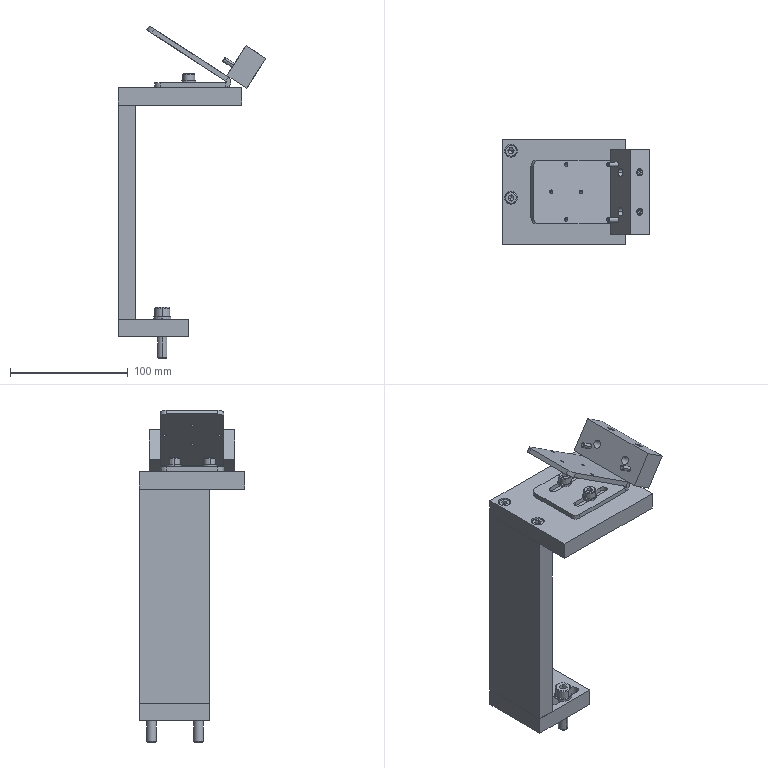Assembly | SolidWorks | mm | 21 component files | 21 solids | 450 faces | box 125.5 x 90 x 282.29 mm | volume 427306 mm3 | plane 252 | cylinder 126 | cone 72 | commonest cylinder face diameters 6 x38 10 x16 7 x12 11 x8 6.6 x8 3.3 x8 8 x8 9 x6
Bill of materials:
AdjustmentPlate | 1 |  | Bent plate bracket in one constant-thickness sheet: a flat base leg and a long inclined leg joined by a tight rounded bend, giving an acute V/stand profile. The inclined leg has four small round holes in a diamond pattern; the base leg has an elongated slot near its free end.
CylinderSupportFrame01 | 1 |  | Square, fairly thick flat plate with two round through holes along one edge and two parallel elongated through slots beside them.
CylinderSupportFrame02 | 1 |  | Tall, slender rectangular bar or block with two small holes in one narrow end face; other faces plain.
CylinderSupportFrame03 | 1 |  | Rectangular flat plate with four through holes: two larger holes near one edge and two smaller holes nearer the middle.
DischargePortPushRodFixingPlate | 1 |  | Rectangular block with two round holes on one long face and, on an adjacent face, two larger round holes plus two smaller counterbored holes. The opposite large face appears plain.
ScrewTAC21-M6-L20(YIHEDA) | 2 |  | Socket-head cap screw shape: cylindrical head with hexagonal socket and chamfered edge, plain cylindrical shank with chamfered tip.
SpringWasherTBN41-6(YIHEDA) | 2 |  | Flat split ring (washer-like annulus) with one radial cut through the ring.
HexSocketHeadCapScrewTAC01-M8-L35(YIHEDA) | 2 |  | Socket-head cap screw shape with hexagonal socket and a relatively longer plain shank with chamfered tip.
SpringWasherTBN41-8(YIHEDA) | 2 |  | Flat split ring with one narrow radial cut; side view shows a thin line at the split.
ScrewTAC21-M4-L25(YIHEDA) | 2 |  | Long socket-head cap screw shape: cylindrical head with hexagonal socket and a long plain cylindrical shank with chamfered/rounded end.
ScrewTAC21-M6-L25(YIHEDA) | 4 |  | Headed pin/screw shape: short cylindrical head with chamfered edges and a long plain cylindrical shank with a chamfered end.
SetScrewTAY12-M6-L12(YIHEDA) | 2 |  | Headless cylindrical set-screw shape with a hexagonal socket at one end and a conical point at the other.
Mates:
1. coincident | CylinderSupportFrame01-1 face at (15.34, 44.766, 58.104) dir (0, 0, 1) | CylinderSupportFrame02-1 face at (0.3404, -45.234, 58.104) dir (0, 0, -1)
2. coincident | CylinderSupportFrame01-1 face at (-44.66, 44.766, 43.104) dir (0, 1, 0) | CylinderSupportFrame02-1 face at (-44.66, 44.766, 38.104) dir (0, 1, 0)
3. coincident | CylinderSupportFrame01-1 face at (0.3404, 44.766, 43.104) dir (-1, 0, 0) | CylinderSupportFrame02-1 face at (0.3404, 44.766, 38.104) dir (-1, 0, 0)
4. coincident | CylinderSupportFrame02-1 face at (0.3404, -45.234, 240.104) dir (0, 0, 1) | CylinderSupportFrame03-1 face at (15.34, 44.766, 240.104) dir (0, 0, -1)
5. coincident | CylinderSupportFrame02-1 face at (-44.66, 44.766, 38.104) dir (0, 1, 0) | CylinderSupportFrame03-1 face at (-44.66, 44.766, 43.104) dir (0, 1, 0)
6. coincident | CylinderSupportFrame02-1 face at (0.3404, 44.766, 38.104) dir (-1, 0, 0) | CylinderSupportFrame03-1 face at (0.3404, 44.766, 43.104) dir (-1, 0, 0)
7. concentric | CylinderSupportFrame01-1 face at (7.84, 34.766, 43.104) dir (0, 0, -1) r 5.5 | ScrewTAC21-M6-L25(YIHEDA)-5 face at (7.84, 34.766, 74.904) dir (0, 0, -1) r 3
8. coincident | CylinderSupportFrame01-1 face at (11.14, 34.766, 49.904) dir (0, 0, -1) | ScrewTAC21-M6-L25(YIHEDA)-5 face at (5.925, 39.385, 49.904) dir (0, 0, 1)
9. concentric | CylinderSupportFrame01-1 face at (7.84, -5.234, 43.104) dir (0, 0, -1) r 5.5 | ScrewTAC21-M6-L25(YIHEDA)-6 face at (7.84, -5.234, 74.904) dir (0, 0, -1) r 3
10. coincident | CylinderSupportFrame01-1 face at (11.14, -5.234, 49.904) dir (0, 0, -1) | ScrewTAC21-M6-L25(YIHEDA)-6 face at (12.565, -6.872, 49.904) dir (0, 0, 1)
11. concentric | CylinderSupportFrame03-1 edge at (7.84, 34.766, 255.104) dir (0, 0, 1) r 5.5 | ScrewTAC21-M6-L25(YIHEDA)-7 face at (7.84, 34.766, 223.304) dir (0, 0, 1) r 3
12. coincident | CylinderSupportFrame03-1 edge at (7.84, 34.766, 248.304) dir (0, 0, 1) r 5.5 | ScrewTAC21-M6-L25(YIHEDA)-7 face at (10.253, 39.146, 248.304) dir (0, 0, -1)
13. concentric | CylinderSupportFrame03-1 face at (7.84, -5.234, 255.104) dir (0, 0, 1) r 3.3 | ScrewTAC21-M6-L25(YIHEDA)-8 face at (7.84, -5.234, 223.304) dir (0, 0, 1) r 3
14. coincident | CylinderSupportFrame03-1 face at (11.14, -5.234, 248.304) dir (0, 0, 1) | ScrewTAC21-M6-L25(YIHEDA)-8 face at (3.523, -2.712, 248.304) dir (0, 0, -1)
15. coincident | CylinderSupportFrame03-1 face at (0.3404, 44.766, 255.104) dir (0, 0, 1) | AdjustmentPlate-1 face at (66.34, -0.234, 255.104) dir (0, 0, -1)
16. parallel | CylinderSupportFrame03-1 face at (-44.66, 44.766, 43.104) dir (0, 1, 0) | AdjustmentPlate-1 face at (101.34, 26.766, 255.104) dir (0, 1, 0)
17. width | AdjustmentPlate-1 face at (101.34, 26.766, 255.104) dir (0, 1, 0) | AdjustmentPlate-1 face at (101.34, -27.234, 255.104) dir (0, -1, 0) | CylinderSupportFrame03-1 face at (-44.66, -45.234, 43.104) dir (0, -1, 0) | CylinderSupportFrame03-1 face at (-44.66, 44.766, 43.104) dir (0, 1, 0)
18. concentric | CylinderSupportFrame03-1 face at (60.34, 14.766, 255.104) dir (0, 0, 1) r 3 | ScrewM6-L20AndSpringWasherAssembly-1/ScrewTAC21-M6-L20(YIHEDA)-1 face at (60.34, 14.766, 240.704) dir (0, 0, 1) r 3
19. concentric | CylinderSupportFrame03-1 face at (60.34, -15.234, 255.104) dir (0, 0, 1) r 3 | ScrewM6-L20AndSpringWasherAssembly-2/ScrewTAC21-M6-L20(YIHEDA)-1 face at (60.34, -15.234, 240.704) dir (0, 0, 1) r 3
20. distance | AdjustmentPlate-1 face at (31.34, -27.234, 255.104) dir (-1, 0, 0) | CylinderSupportFrame03-1 face at (0.3404, 44.766, 43.104) dir (-1, 0, 0)
21. concentric | DischargePortPushRodFixingPlate-1 face at (114.95, -23.884, 262.904) dir (0.8387, 0, -0.5446) r 4 | ScrewTAC21-M4-L25(YIHEDA)-1 face at (90.126, -23.884, 279.026) dir (0.8387, 0, -0.5446) r 2
22. coincident | DischargePortPushRodFixingPlate-1 face at (111.092, -26.134, 265.41) dir (0.8387, 0, -0.5446) | ScrewTAC21-M4-L25(YIHEDA)-1 face at (109.238, -24.698, 262.555) dir (-0.8387, 0, 0.5446)
23. concentric | DischargePortPushRodFixingPlate-1 face at (117.457, -17.134, 285.125) dir (0.5446, 0, 0.8387) r 3 | SetScrewTAY12-M6-L12(YIHEDA)-1 face at (110.921, -17.134, 275.061) dir (0.5446, 0, 0.8387) r 3
24. coincident | DischargePortPushRodFixingPlate-1 face at (125.843, 35.916, 279.678) dir (0.5446, 0, 0.8387) | SetScrewTAY12-M6-L12(YIHEDA)-1 face at (117.457, -17.134, 285.125) dir (0.5446, 0, 0.8387)
25. tangent | CylinderSupportFrame01-1 face at (50.34, -9.734, 43.104) dir (0, 1, 0) | ScrewM8-L35AndSpringWasherAssembly-1/HexSocketHeadCapScrewTAC01-M8-L35(YIHEDA)-1 face at (37.83, -5.734, 25.104) dir (0, 0, 1) r 4
26. distance | CylinderSupportFrame01-1 face at (25.34, -5.234, 43.104) dir (0, 0, 1) r 4.5 | ScrewM8-L35AndSpringWasherAssembly-1/HexSocketHeadCapScrewTAC01-M8-L35(YIHEDA)-1 face at (37.83, -5.734, 25.104) dir (0, 0, 1) r 4
27. coincident | CylinderSupportFrame01-1 face at (15.34, 44.766, 58.104) dir (0, 0, 1) | ScrewM8-L35AndSpringWasherAssembly-1/SpringWasherTBN41-8(YIHEDA)-1 face at (37.83, -5.734, 58.104) dir (0, 0, -1)
28. tangent | CylinderSupportFrame01-1 face at (50.34, 30.266, 43.104) dir (0, 1, 0) | ScrewM8-L35AndSpringWasherAssembly-2/HexSocketHeadCapScrewTAC01-M8-L35(YIHEDA)-1 face at (37.83, 34.266, 25.104) dir (0, 0, 1) r 4
29. coincident | ScrewM8-L35AndSpringWasherAssembly-1/HexSocketHeadCapScrewTAC01-M8-L35(YIHEDA)-1 face at (37.83, -5.734, 68.104) dir (0, 0, 1) | ScrewM8-L35AndSpringWasherAssembly-2/HexSocketHeadCapScrewTAC01-M8-L35(YIHEDA)-1 face at (37.83, 34.266, 68.104) dir (0, 0, 1)
30. distance | CylinderSupportFrame01-1 face at (25.34, 34.766, 43.104) dir (0, 0, 1) r 4.5 | ScrewM8-L35AndSpringWasherAssembly-2/HexSocketHeadCapScrewTAC01-M8-L35(YIHEDA)-1 face at (37.83, 34.266, 60.104) dir (0, 0, 1) r 6.5
31. concentric | ScrewTAC21-M6-L20(YIHEDA)-1 face at (15.436, 12.399, 4.727) dir (0, 0, 1) r 3 | SpringWasherTBN41-6(YIHEDA)-1 face at (15.436, 12.399, 24.727) dir (0, 0, 1) r 3.05
32. coincident | ScrewTAC21-M6-L20(YIHEDA)-1 face at (15.436, 17.399, 24.727) dir (0, 0, -1) | SpringWasherTBN41-6(YIHEDA)-1 face at (15.436, 12.399, 24.727) dir (0, 0, 1)
33. concentric | HexSocketHeadCapScrewTAC01-M8-L35(YIHEDA)-1 face at (4.221, 1.897, 21.5) dir (0, 0, 1) r 4 | SpringWasherTBN41-8(YIHEDA)-1 face at (4.221, 1.897, 56.5) dir (0, 0, 1) r 4.05
34. coincident | HexSocketHeadCapScrewTAC01-M8-L35(YIHEDA)-1 face at (4.221, 8.397, 56.5) dir (0, 0, -1) | SpringWasherTBN41-8(YIHEDA)-1 face at (4.221, 1.897, 56.5) dir (0, 0, 1)